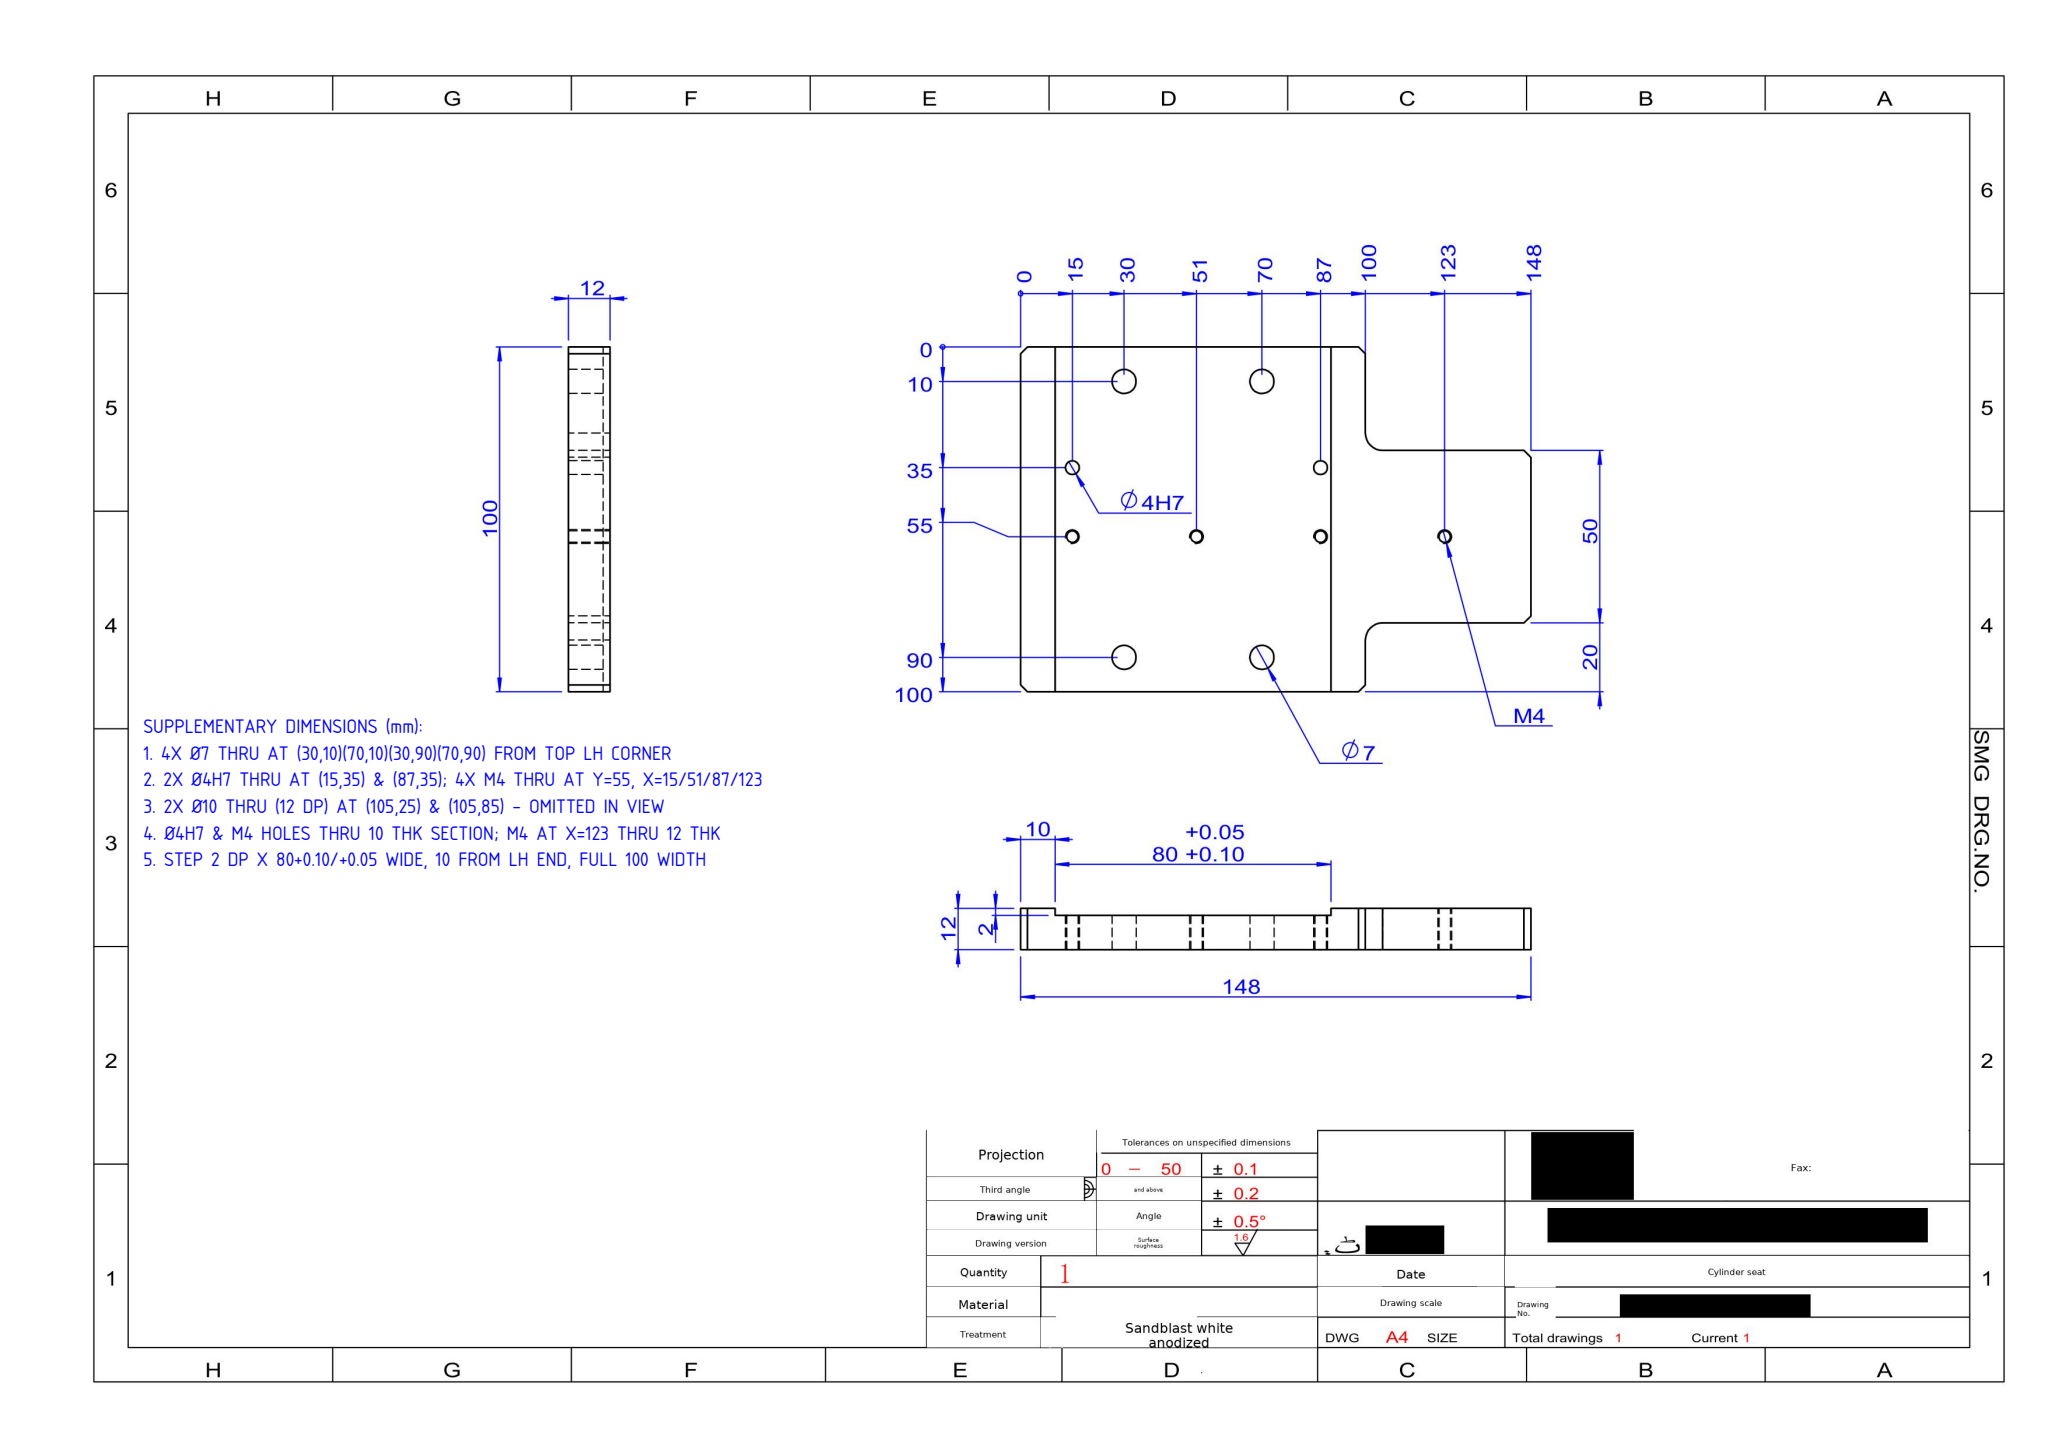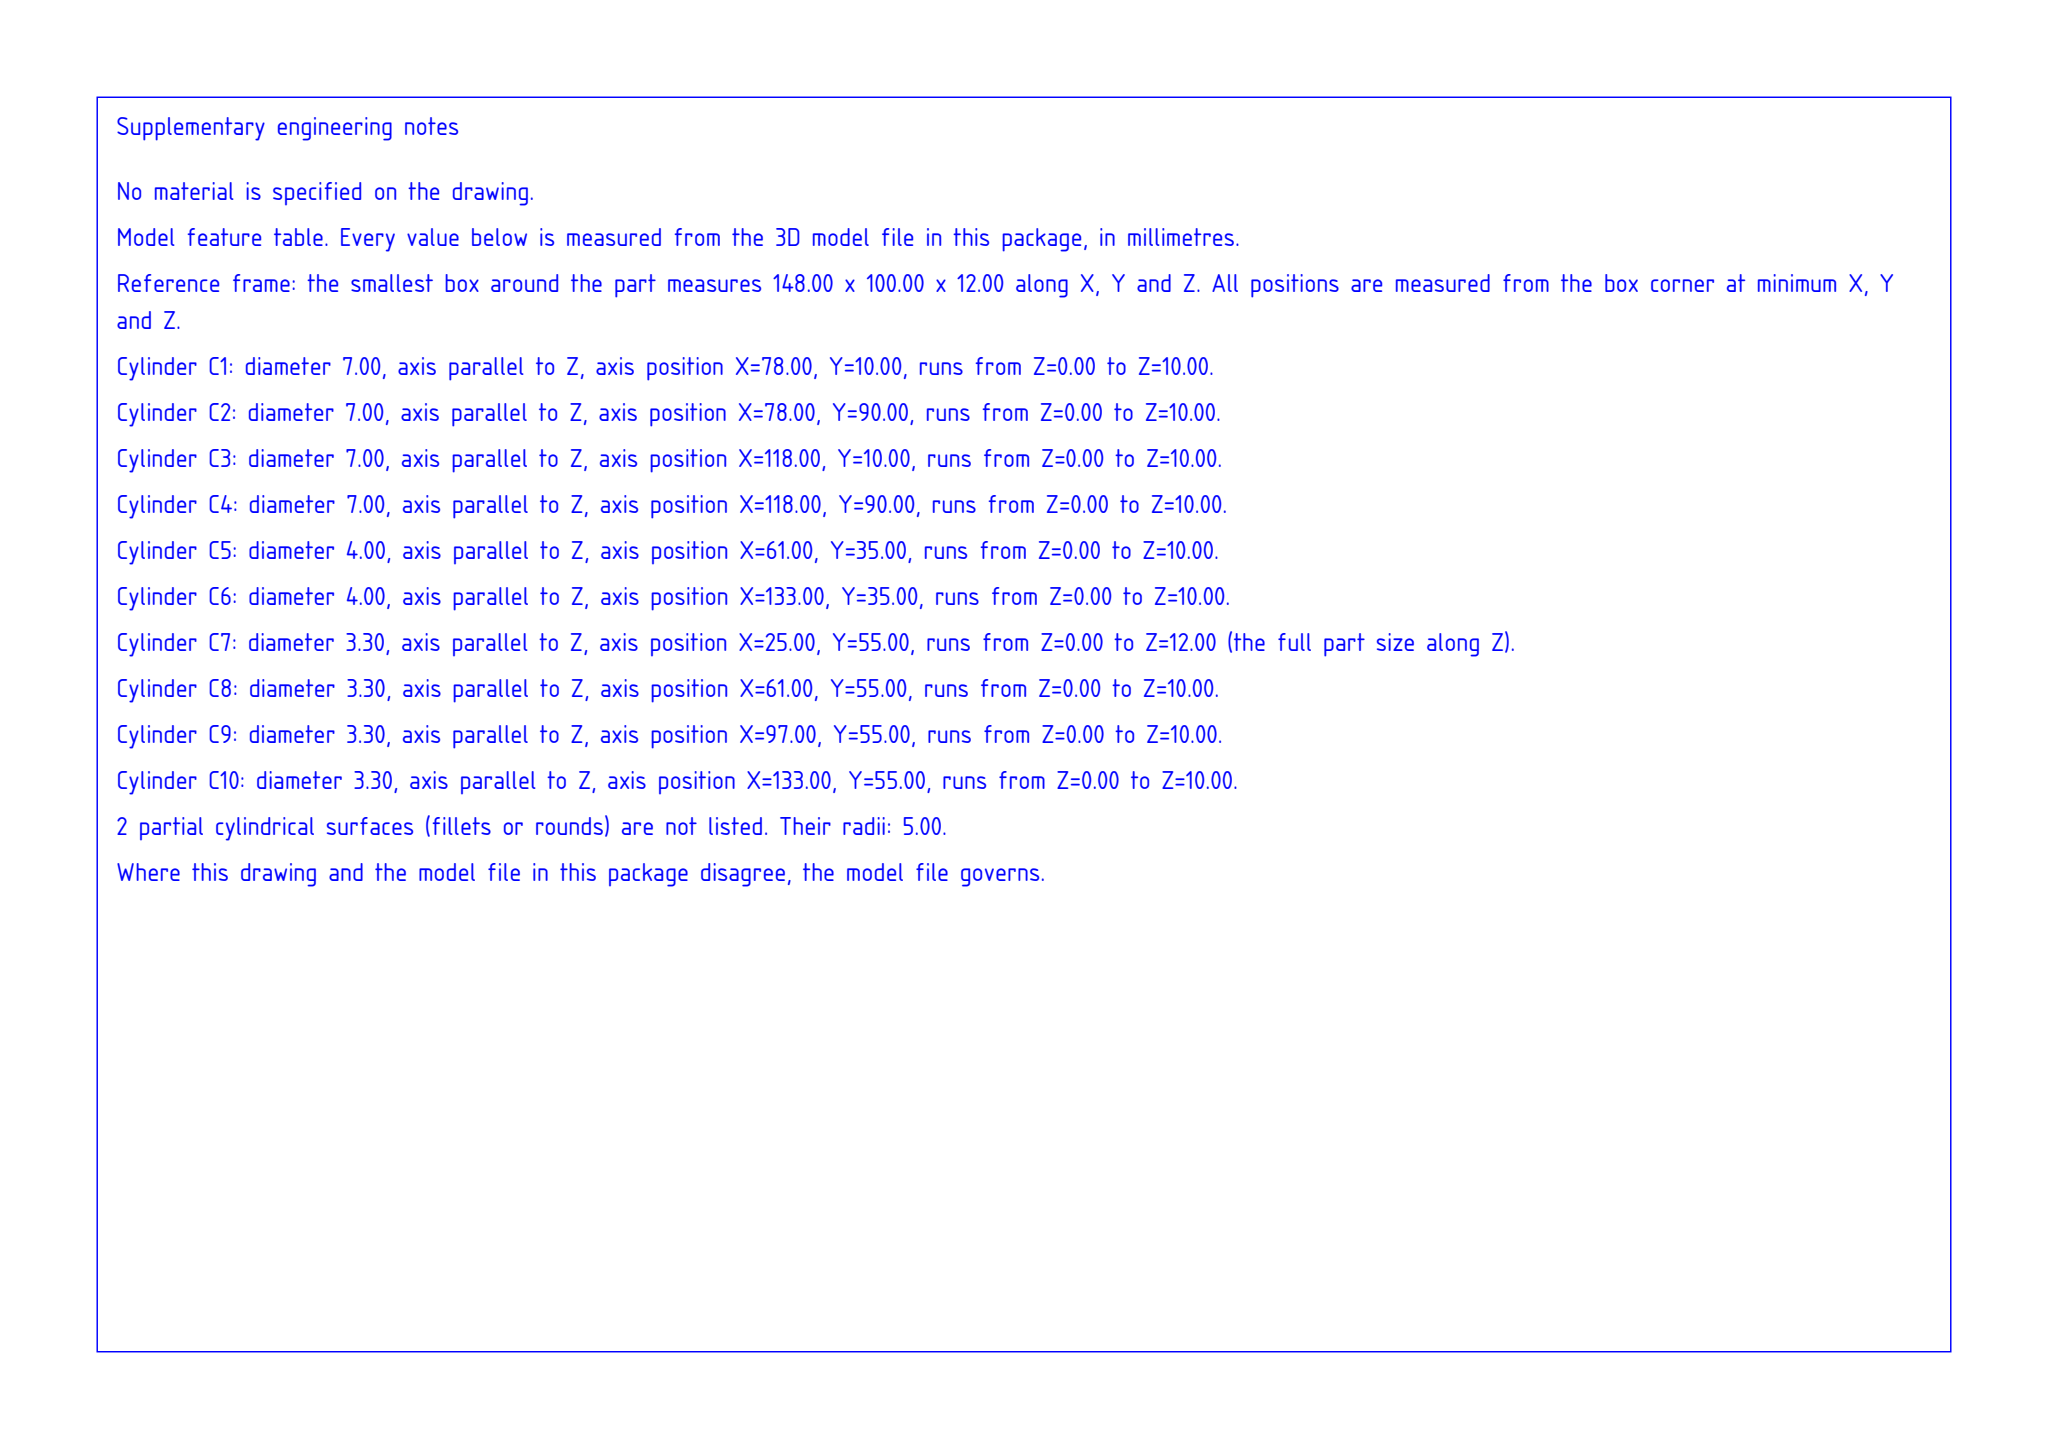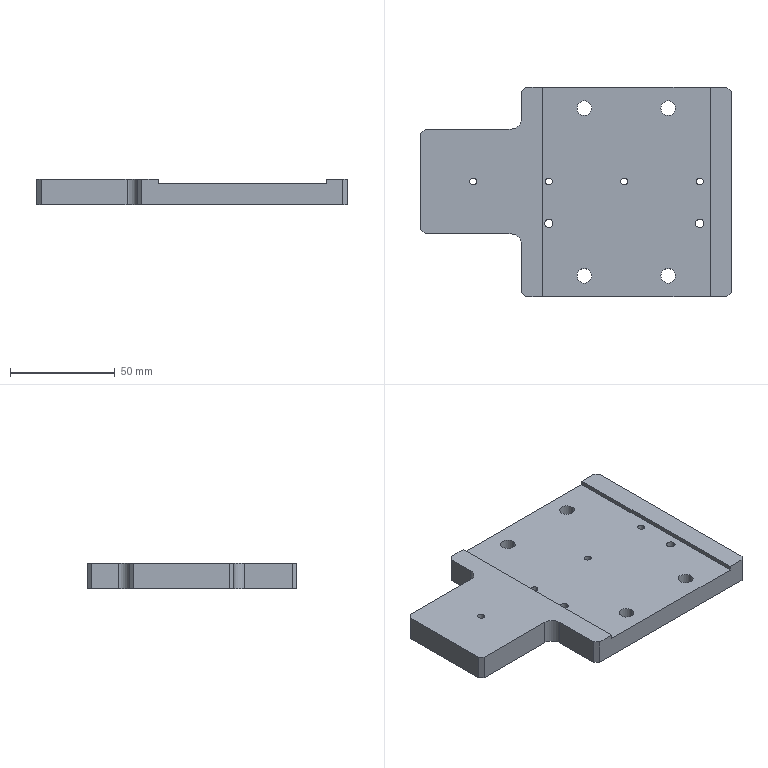Part | SolidWorks | mm | 1 solid | 42 faces | box 148 x 100 x 12 mm | volume 130635 mm3 | cylinder 22 | plane 20 | commonest cylinder face diameters 3.3 x8 7 x8 4 x4 10 x2